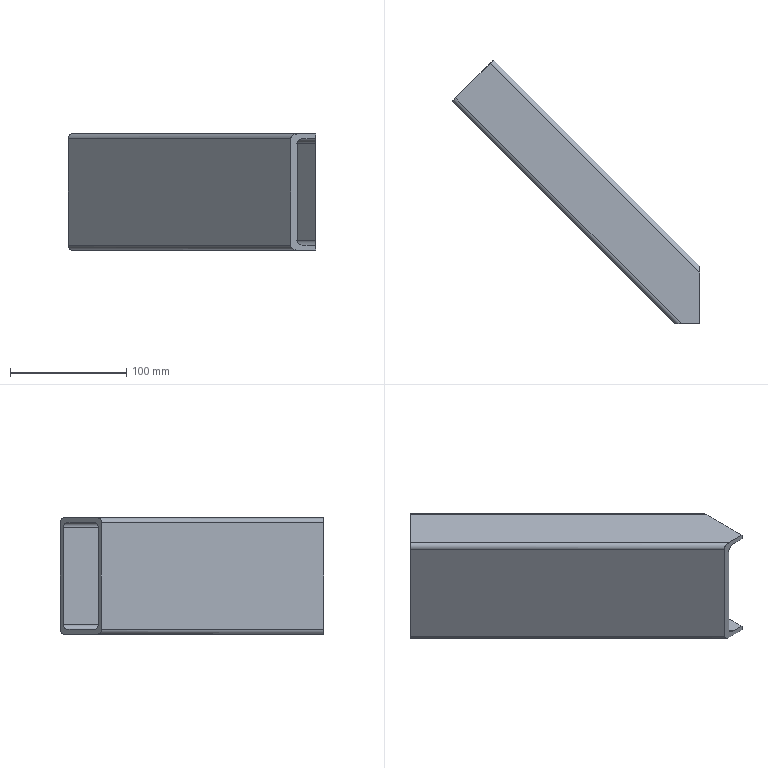Component | NX | BASE_FRAME_RECT_TUBE3 | 1 solid | 19 faces | volume 302256 mm3 | plane 11 | cylinder 8 | commonest cylinder face diameters 8 x8